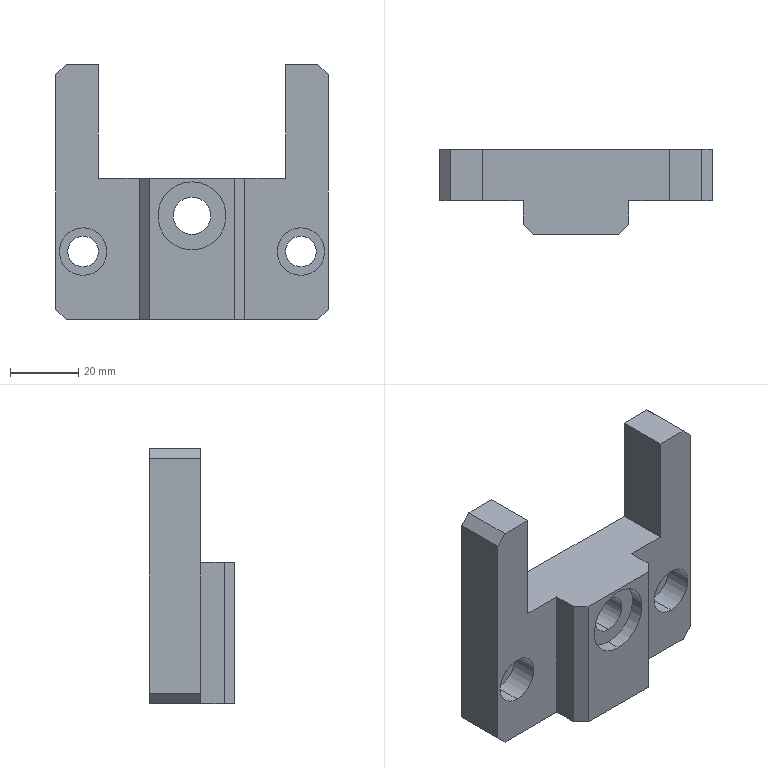Component | SolidWorks | RisingCylinderOutputPlate-1 | 1 solid | 38 faces | box 80 x 25 x 75 mm | volume 66527 mm3 | plane 24 | cylinder 14 | commonest cylinder face diameters 14 x4 9 x4 17 x2 11 x2 20 x2
build123d program:
from build123d import *

# Parameters (mm, degrees)
SKETCH1_W                                  = 80
SKETCH1_H                                  = 80
BOSS_EXTRUDE1_DEPTH                        = 15
SKETCH2_W                                  = 55
SKETCH2_H                                  = 27.5
CUT_EXTRUDE1_DEPTH                         = 59.523
M10_HEX_HEAD_BOLT_COUNTERBORE1_D           = 11
M10_HEX_HEAD_BOLT_COUNTERBORE1_CBORE_D     = 17
M10_HEX_HEAD_BOLT_COUNTERBORE1_CBORE_DEPTH = 11
SKETCH5_R                                  = 8
CUT_EXTRUDE2_DEPTH                         = 3
BOSS_EXTRUDE2_START                        = 12
SKETCH6_W                                  = 80
SKETCH6_H                                  = 52.5
SKETCH6_R                                  = 8
BOSS_EXTRUDE2_DEPTH                        = 12
BOSS_EXTRUDE3_START                        = 12
SKETCH7_R                                  = 8
SKETCH7_R_2                                = 5.5
BOSS_EXTRUDE3_DEPTH                        = 12
SKETCH8_W                                  = 12.5
SKETCH8_H                                  = 12
CUT_EXTRUDE3_DEPTH                         = 68.685
SKETCH9_W                                  = 12
SKETCH9_H                                  = 52.5
CUT_EXTRUDE4_DEPTH                         = 12
SKETCH10_W                                 = 31
SKETCH10_H                                 = 1
CUT_EXTRUDE5_DEPTH                         = 91.692
SKETCH11_W                                 = 80
SKETCH11_H                                 = 12
CUT_EXTRUDE6_DEPTH                         = 63.258
SKETCH12_W                                 = 12.5
SKETCH12_H                                 = 15
BOSS_EXTRUDE4_DEPTH                        = 7
M8_HEX_HEAD_BOLT_COUNTERBORE1_D            = 9
M8_HEX_HEAD_BOLT_COUNTERBORE1_DEPTH        = 19.75
M8_HEX_HEAD_BOLT_COUNTERBORE1_CBORE_D      = 14
M8_HEX_HEAD_BOLT_COUNTERBORE1_CBORE_DEPTH  = 8
M8_HEX_HEAD_BOLT_COUNTERBORE1_TIP          = 2.704
CHAMFER1_SIZE                              = 3
BOSS_EXTRUDE5_DEPTH                        = 1
SKETCH16_R                                 = 10
CUT_EXTRUDE7_DEPTH                         = 5
SKETCH17_W                                 = 31
SKETCH17_H                                 = 41.5
CUT_EXTRUDE8_DEPTH                         = 1
CHAMFER2_SIZE                              = 3


with BuildPart() as part:
    # Sketch1 → Boss-Extrude1 (new body)
    with BuildSketch(Plane(origin=(0, 0, 0), x_dir=(1, 0, 0), z_dir=(0, 1, 0))):
        Rectangle(SKETCH1_W, SKETCH1_H)
    extrude(amount=BOSS_EXTRUDE1_DEPTH)

    # Sketch2 → Cut-Extrude1 (cut, through all)
    with BuildSketch(Plane(origin=(0, 15, 0), x_dir=(1, 0, 0), z_dir=(0, 1, 0))):
        with Locations((0, 26.25)):
            Rectangle(SKETCH2_W, SKETCH2_H)
    extrude(amount=-CUT_EXTRUDE1_DEPTH, mode=Mode.SUBTRACT)

    # M10 Hex Head Bolt Counterbore1 (through all)
    with Locations(Plane(origin=(0, 15, 0), x_dir=(1, 0, 0), z_dir=(0, 1, 0))):
        with Locations((0, 2.5)):
            CounterBoreHole(M10_HEX_HEAD_BOLT_COUNTERBORE1_D / 2, M10_HEX_HEAD_BOLT_COUNTERBORE1_CBORE_D / 2, M10_HEX_HEAD_BOLT_COUNTERBORE1_CBORE_DEPTH)

    # Sketch5 → Cut-Extrude2 (cut)
    with BuildSketch(Plane.XZ):
        with Locations(Location((0, -2.5, 0), (0, 0, 270))):
            Circle(SKETCH5_R)
    extrude(amount=-CUT_EXTRUDE2_DEPTH, mode=Mode.SUBTRACT)

    # Sketch6 → Boss-Extrude2 (add)
    with BuildSketch(Plane.XZ.offset(BOSS_EXTRUDE2_START)):
        with Locations((0, 13.75)):
            Rectangle(SKETCH6_W, SKETCH6_H)
        with Locations(Location((0, -2.5, 0), (0, 0, 270))):
            Circle(SKETCH6_R, mode=Mode.SUBTRACT)
    extrude(amount=-BOSS_EXTRUDE2_DEPTH)

    # Sketch7 → Boss-Extrude3 (add)
    with BuildSketch(Plane.XZ.offset(-3).offset(BOSS_EXTRUDE3_START)):
        with Locations(Location((0, -2.5, 0), (0, 0, 270))):
            Circle(SKETCH7_R)
        with Locations(Location((0, -2.5, 0), (0, 0, 90))):
            Circle(SKETCH7_R_2, mode=Mode.SUBTRACT)
    extrude(amount=-BOSS_EXTRUDE3_DEPTH)

    # Sketch8 → Cut-Extrude3 (cut, through all)
    with BuildSketch(Plane(origin=(0, 0, -12.5), x_dir=(-1, 0, 0), z_dir=(0, 0, -1))):
        with Locations((-33.75, -6)):
            Rectangle(SKETCH8_W, SKETCH8_H)
        with Locations((33.75, -6)):
            Rectangle(SKETCH8_W, SKETCH8_H)
    extrude(amount=-CUT_EXTRUDE3_DEPTH, mode=Mode.SUBTRACT)

    # Sketch9 → Cut-Extrude4 (cut)
    with BuildSketch(Plane.XZ.offset(12)):
        with Locations((-21.5, 13.75)):
            Rectangle(SKETCH9_W, SKETCH9_H)
    cut_extrude4 = extrude(amount=-CUT_EXTRUDE4_DEPTH, mode=Mode.SUBTRACT)

    # Mirror1: Cut-Extrude4 across plane
    add(cut_extrude4.mirror(Plane(origin=(0, 0, 0), x_dir=(0, 0, 1), z_dir=(1, 0, 0))), mode=Mode.SUBTRACT)

    # Sketch10 → Cut-Extrude5 (cut, through all)
    with BuildSketch(Plane.XY.offset(40)):
        with Locations((0, -11.5)):
            Rectangle(SKETCH10_W, SKETCH10_H)
    extrude(amount=-CUT_EXTRUDE5_DEPTH, mode=Mode.SUBTRACT)

    # Sketch11 → Cut-Extrude6 (cut, through all)
    with BuildSketch(Plane(origin=(0, 15, 0), x_dir=(1, 0, 0), z_dir=(0, 1, 0))):
        with Locations((0, -34)):
            Rectangle(SKETCH11_W, SKETCH11_H)
    extrude(amount=-CUT_EXTRUDE6_DEPTH, mode=Mode.SUBTRACT)

    # Sketch12 → Boss-Extrude4 (add)
    with BuildSketch(Plane(origin=(0, 0, -40), x_dir=(-1, 0, 0), z_dir=(0, 0, -1))):
        with Locations((-33.75, 7.5)):
            Rectangle(SKETCH12_W, SKETCH12_H)
        with Locations((33.75, 7.5)):
            Rectangle(SKETCH12_W, SKETCH12_H)
    extrude(amount=BOSS_EXTRUDE4_DEPTH)

    # M8 Hex Head Bolt Counterbore1
    with Locations(Plane(origin=(0, 0, 0), x_dir=(-1, 0, 0), z_dir=(0, -1, 0))):
        with Locations((32, -8), (-32, -8)):
            CounterBoreHole(M8_HEX_HEAD_BOLT_COUNTERBORE1_D / 2, M8_HEX_HEAD_BOLT_COUNTERBORE1_CBORE_D / 2, M8_HEX_HEAD_BOLT_COUNTERBORE1_CBORE_DEPTH, depth=M8_HEX_HEAD_BOLT_COUNTERBORE1_DEPTH)
            with Locations((0, 0, -(M8_HEX_HEAD_BOLT_COUNTERBORE1_DEPTH + M8_HEX_HEAD_BOLT_COUNTERBORE1_TIP / 2))):  # 118° drill point
                Cone(0, M8_HEX_HEAD_BOLT_COUNTERBORE1_D / 2, M8_HEX_HEAD_BOLT_COUNTERBORE1_TIP, mode=Mode.SUBTRACT)

    # Chamfer1
    chamfer1_edges = [part.edges().sort_by_distance(p)[0] for p in [
        (-40, 7.5, 28),
        (40, 7.5, 28),
        (40, 7.5, -47),
        (-40, 7.5, -47),
    ]]
    chamfer(chamfer1_edges, length=CHAMFER1_SIZE)

    # Sketch15 → Boss-Extrude5 (add)
    with BuildSketch(Plane(origin=(0, 0, -12.5), x_dir=(-1, 0, 0), z_dir=(0, 0, -1))):
        Polygon((-15.5, 0), (-15.5, -11), (15.5, -11), (15.5, 0), (27.5, 0), (27.5, 15), (-27.5, 15), (-27.5, 0), align=None)
    extrude(amount=BOSS_EXTRUDE5_DEPTH)

    # Sketch16 → Cut-Extrude7 (cut)
    with BuildSketch(Plane.XZ.offset(11)):
        with Locations(Location((0, -2.5, 0), (0, 0, 270))):
            Circle(SKETCH16_R)
    extrude(amount=-CUT_EXTRUDE7_DEPTH, mode=Mode.SUBTRACT)

    # Sketch17 → Cut-Extrude8 (cut)
    with BuildSketch(Plane.XZ.offset(11)):
        with Locations((0, 7.25)):
            Rectangle(SKETCH17_W, SKETCH17_H)
    extrude(amount=-CUT_EXTRUDE8_DEPTH, mode=Mode.SUBTRACT)

    # Chamfer2
    chamfer2_edges = [part.edges().sort_by_distance(p)[0] for p in [
        (-15.5, -10, 7.25),
        (15.5, -10, 7.25),
    ]]
    chamfer(chamfer2_edges, length=CHAMFER2_SIZE)


solid = part.part

# Placed as in the assembly
solid = solid.moved(Location((-29.507, -43.411, 428), (-180, 0, 180)))